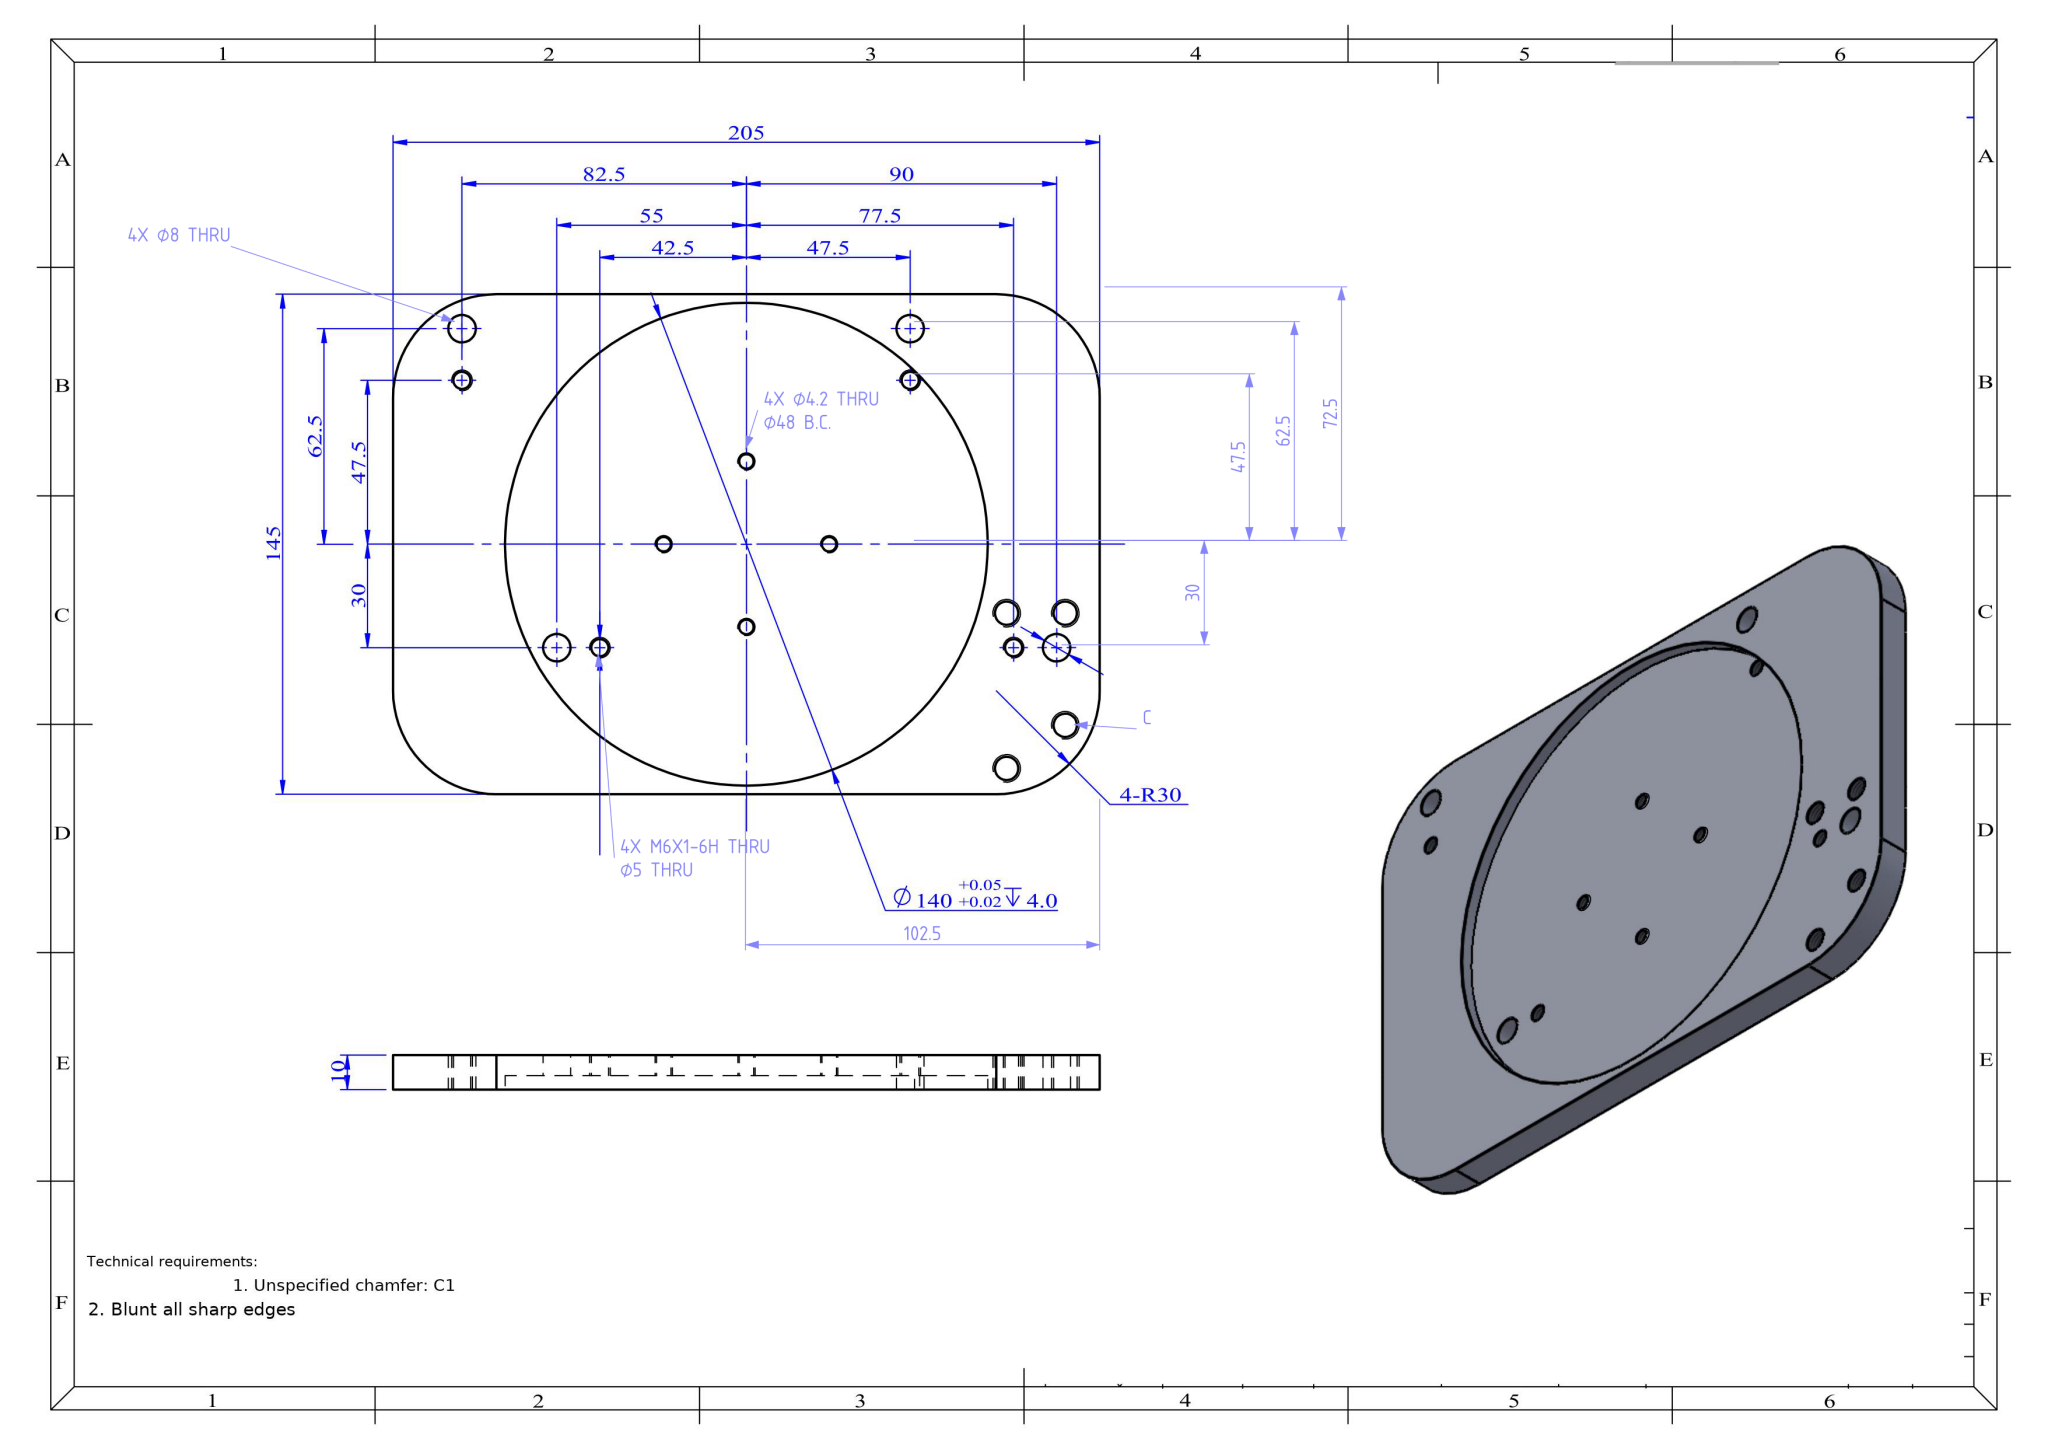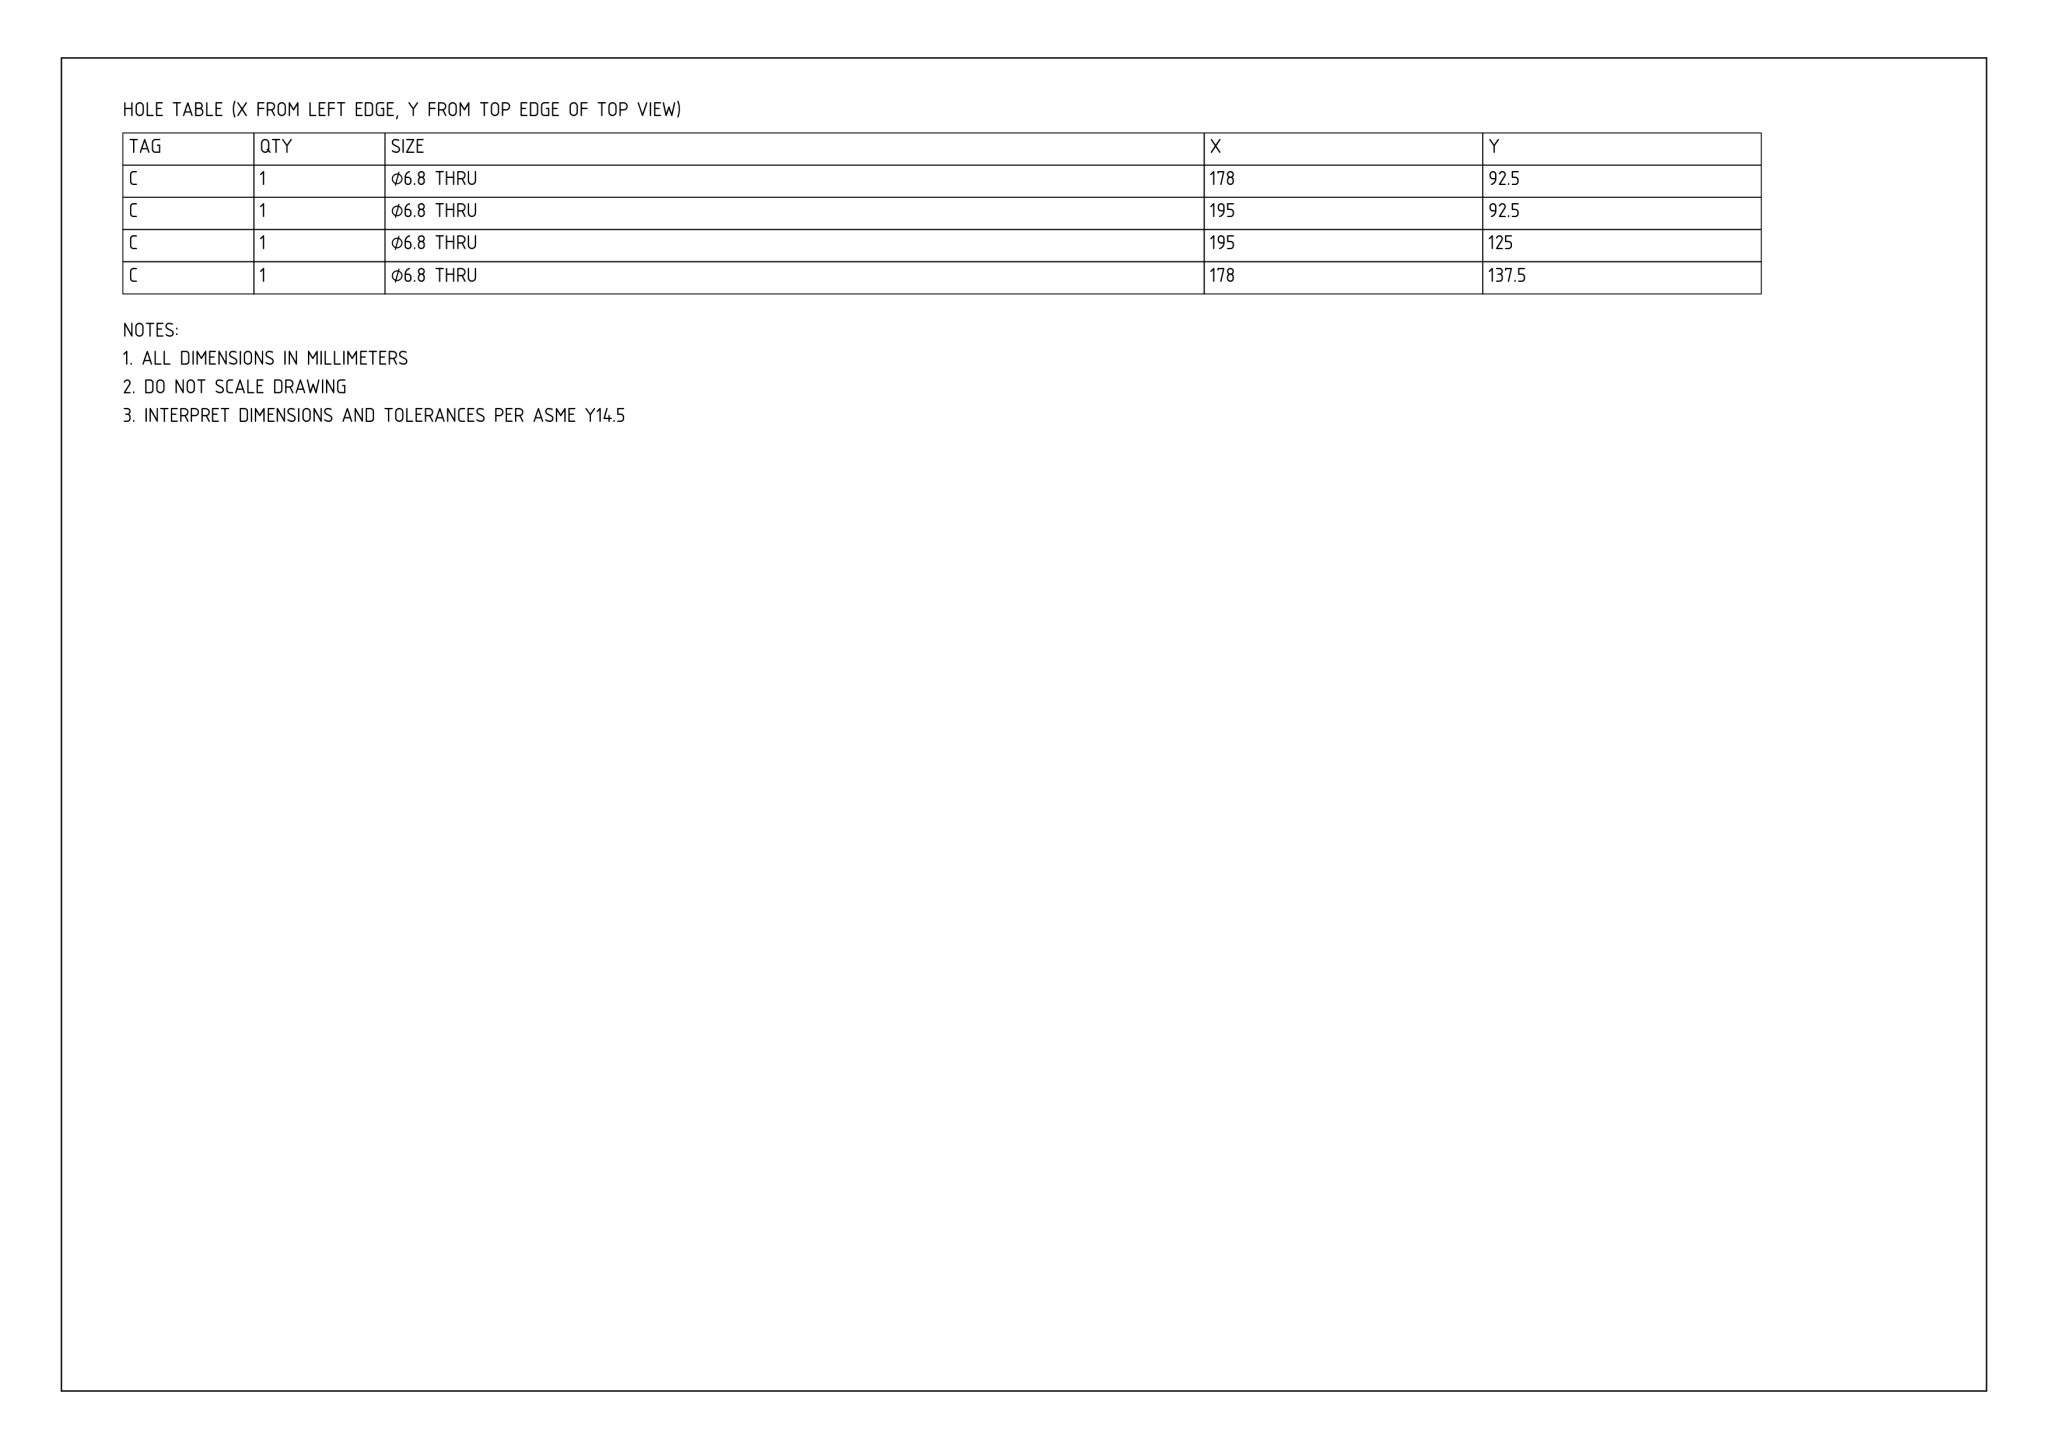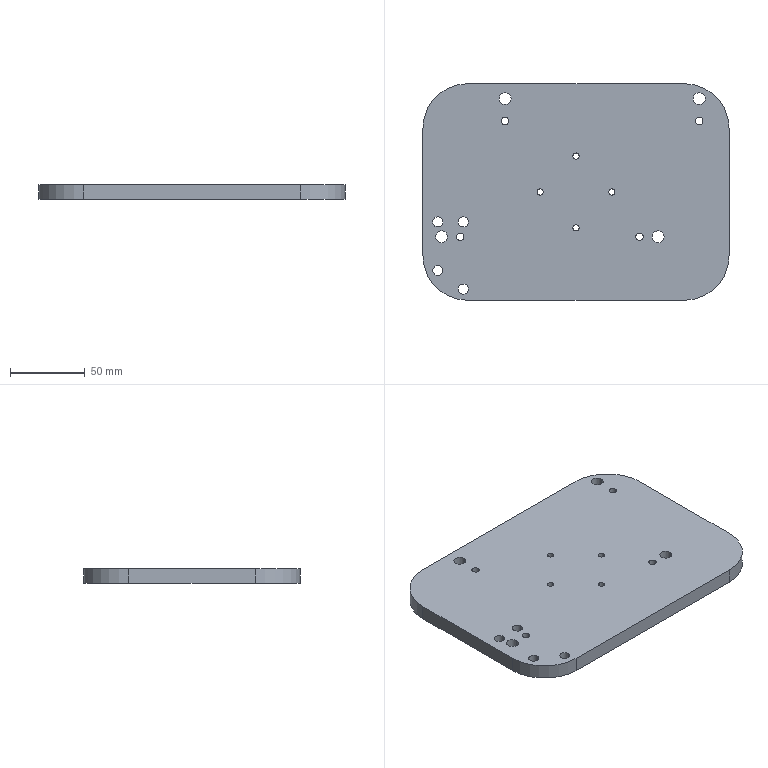Part | NX | mm | 1 solid | 45 faces | box 205 x 145 x 10 mm | volume 223726 mm3 | cylinder 38 | plane 7 | commonest cylinder face diameters 4.2 x8 6.8 x8 5 x8 8 x8 60 x4 140 x2